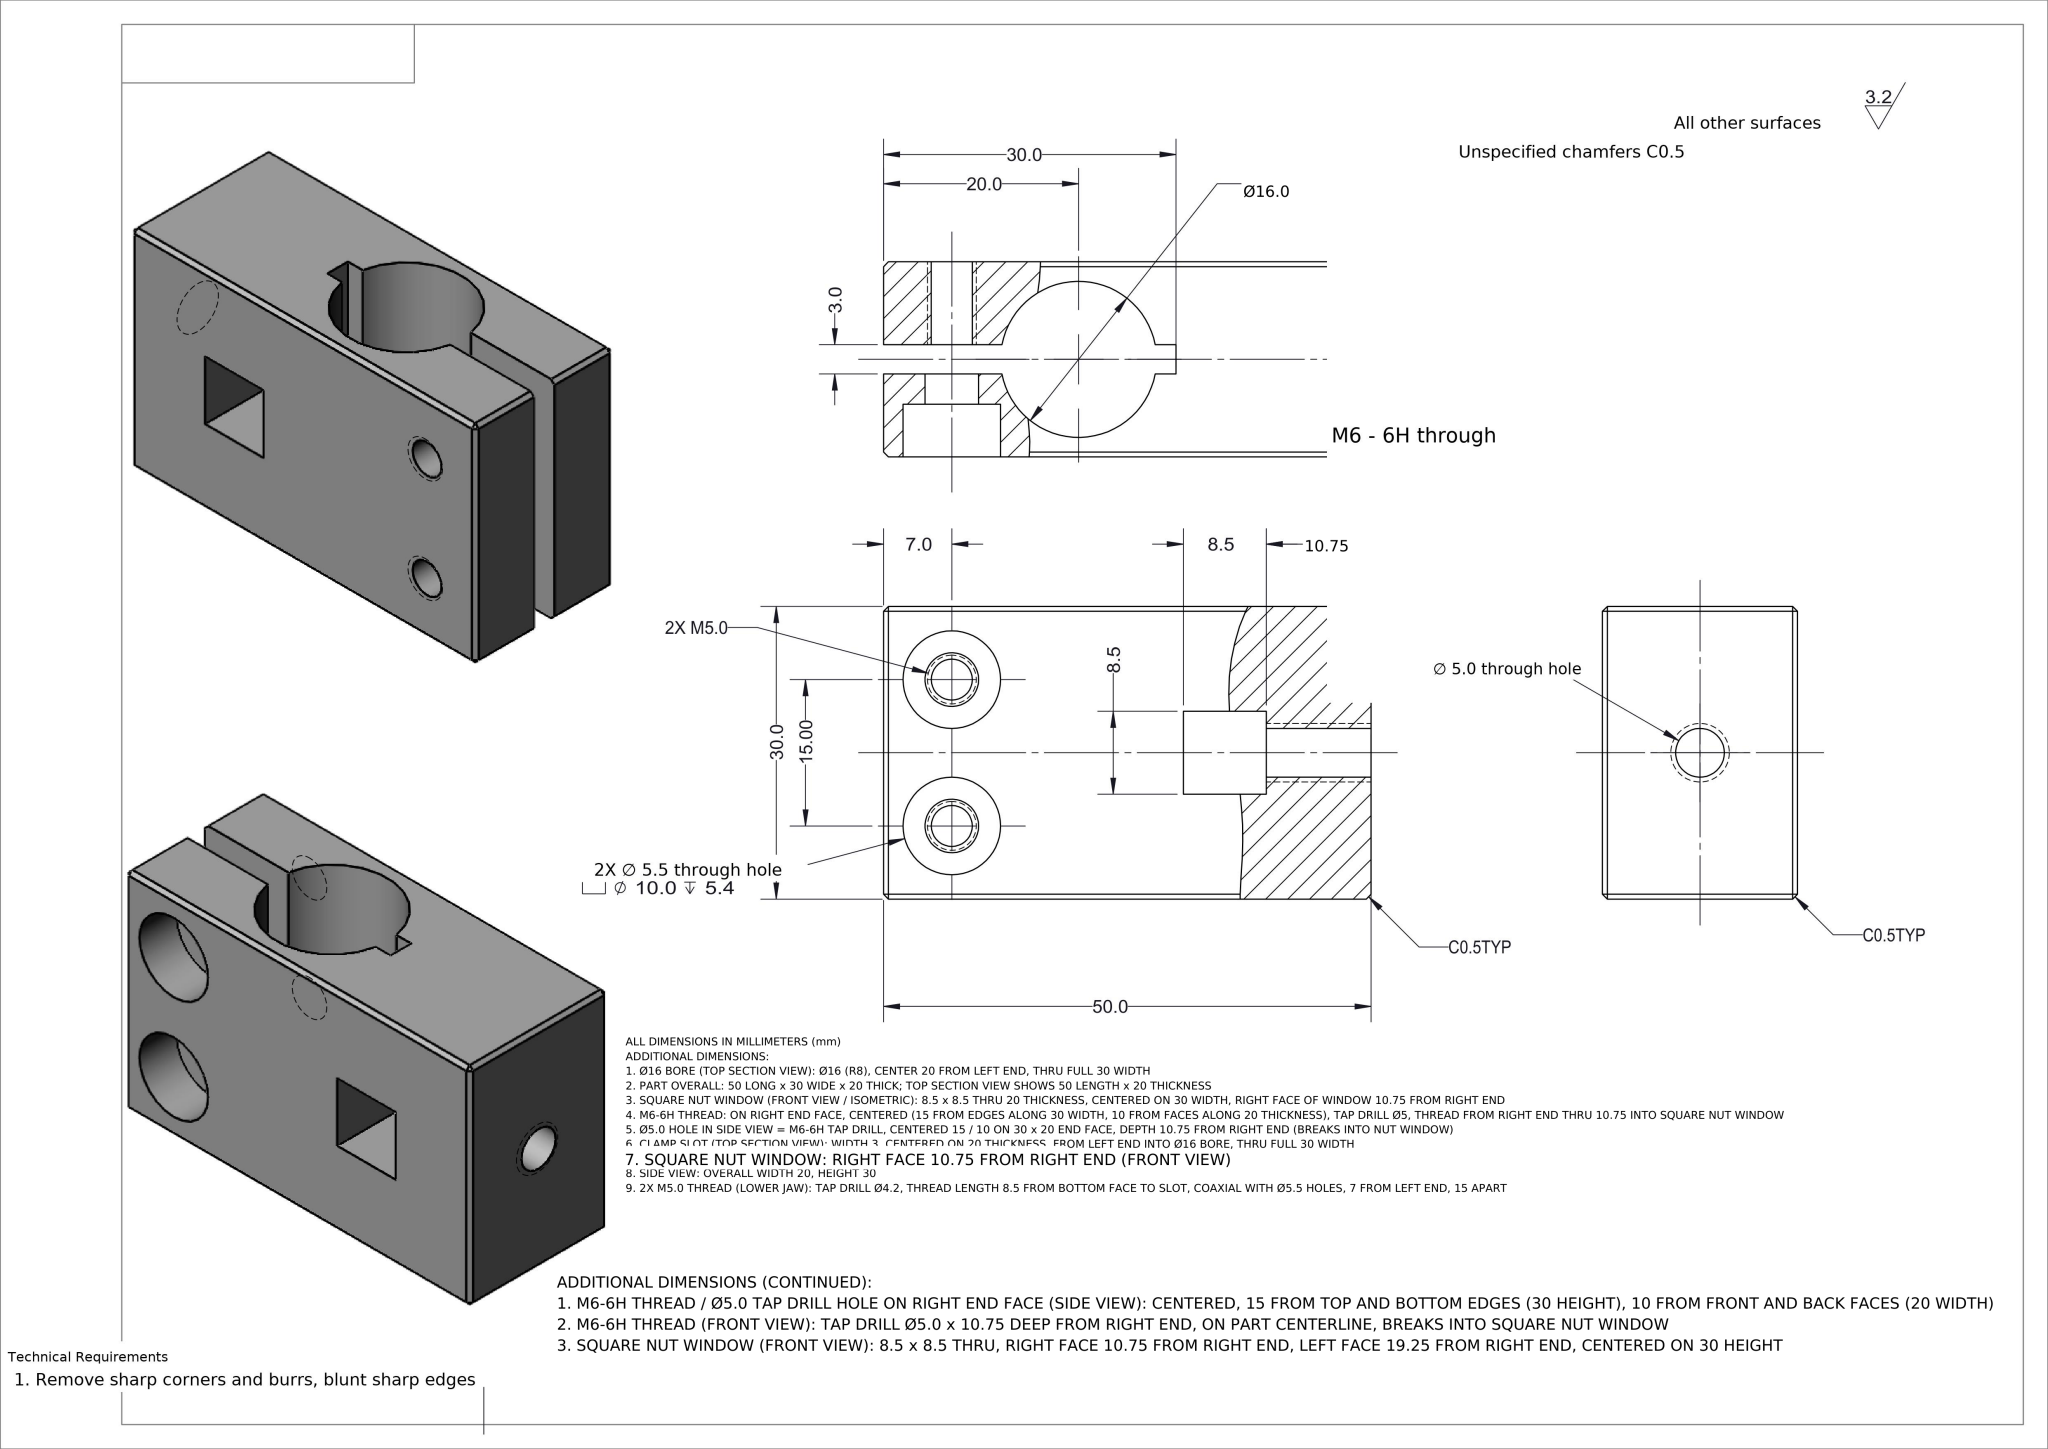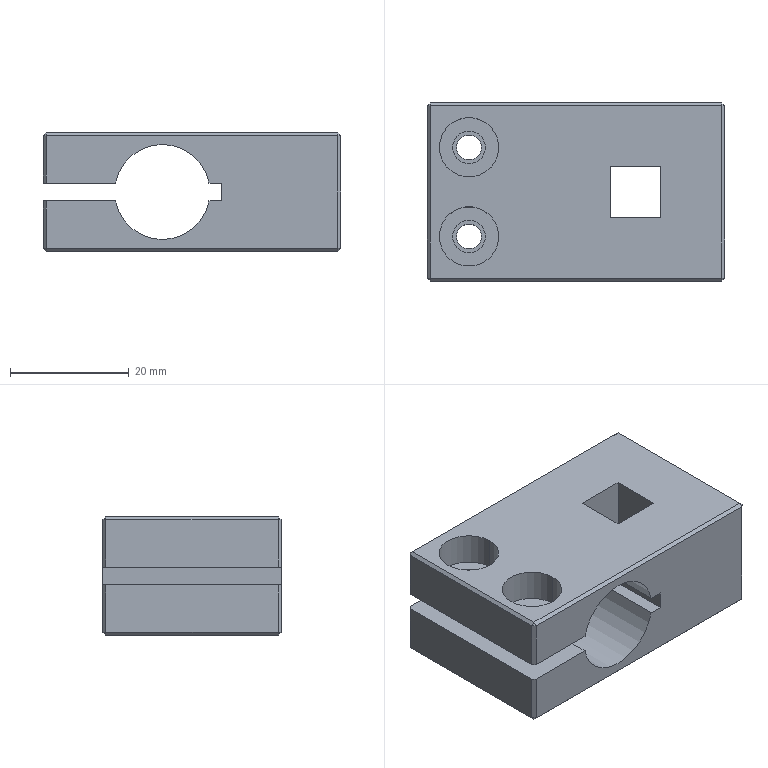Part | NX | mm | 1 solid | 56 faces | box 50 x 30 x 20 mm | volume 19764 mm3 | plane 40 | cylinder 16 | commonest cylinder face diameters 4.2 x4 10 x4 5.5 x4 5 x2 16 x2